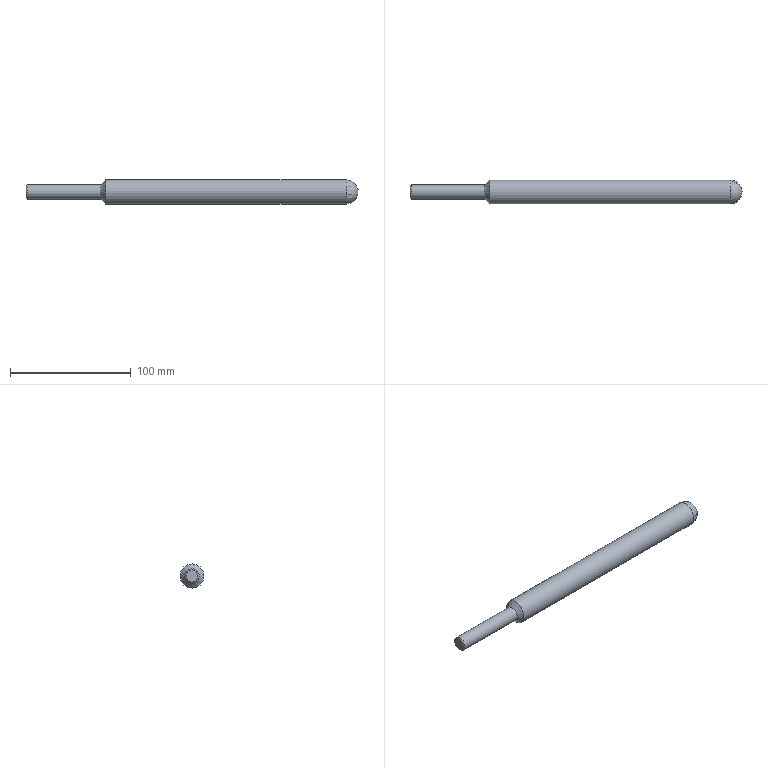Component | NX | TOMMY_BAR | 1 solid | 6 faces | box 275 x 20 x 20 mm | volume 72427 mm3 | cylinder 2 | cone 2 | plane 1 | sphere 1 | commonest cylinder face diameters 12 x1 20 x1
STEP:
#1=CARTESIAN_POINT('',(0.,0.,0.));
#2=DIRECTION('',(0.,0.,1.));
#3=DIRECTION('',(1.,0.,0.));
#4=AXIS2_PLACEMENT_3D('',#1,#2,#3);
#5=CARTESIAN_POINT('',(-19.,240.,259.5));
#6=VERTEX_POINT('',#5);
#7=CARTESIAN_POINT('',(-19.,246.,265.5));
#8=VERTEX_POINT('',#7);
#9=CARTESIAN_POINT('',(-19.,240.,265.5));
#10=DIRECTION('',(1.,0.,0.));
#11=DIRECTION('',(0.,0.,-1.));
#12=AXIS2_PLACEMENT_3D('',#9,#10,#11);
#13=CIRCLE('',#12,6.);
#14=CARTESIAN_POINT('',(42.,240.,265.5));
#15=DIRECTION('',(-1.,0.,0.));
#16=DIRECTION('',(0.,0.,1.));
#17=AXIS2_PLACEMENT_3D('',#14,#15,#16);
#18=CYLINDRICAL_SURFACE('',#17,6.);
#19=CARTESIAN_POINT('',(3.142,61.));
#20=DIRECTION('',(-1.,0.));
#21=VECTOR('',#20,1.);
#22=LINE('',#19,#21);
#23=(GEOMETRIC_REPRESENTATION_CONTEXT(2)PARAMETRIC_REPRESENTATION_CONTEXT()REPRESENTATION_CONTEXT('',''));
#24=DEFINITIONAL_REPRESENTATION('',(#22),#23);
#25=PCURVE('',#18,#24);
#26=CARTESIAN_POINT('',(-19.,240.,265.5));
#27=DIRECTION('',(1.,0.,0.));
#28=DIRECTION('',(0.,0.,-1.));
#29=AXIS2_PLACEMENT_3D('',#26,#27,#28);
#30=CONICAL_SURFACE('',#29,6.,0.7854);
#31=CARTESIAN_POINT('',(0.,0.));
#32=DIRECTION('',(1.,0.));
#33=VECTOR('',#32,1.);
#34=LINE('',#31,#33);
#35=(GEOMETRIC_REPRESENTATION_CONTEXT(2)PARAMETRIC_REPRESENTATION_CONTEXT()REPRESENTATION_CONTEXT('',''));
#36=DEFINITIONAL_REPRESENTATION('',(#34),#35);
#37=PCURVE('',#30,#36);
#38=SURFACE_CURVE('',#13,(#25,#37),.PCURVE_S1.);
#39=EDGE_CURVE('',#6,#8,#38,.T.);
#40=ORIENTED_EDGE('',*,*,#39,.T.);
#41=CARTESIAN_POINT('',(42.,246.,265.5));
#42=VERTEX_POINT('',#41);
#43=CARTESIAN_POINT('',(42.,246.,265.5));
#44=CARTESIAN_POINT('',(-19.,246.,265.5));
#45=B_SPLINE_CURVE_WITH_KNOTS('',1,(#43,#44),.UNSPECIFIED.,.F.,.F.,(2,2),(0.,61.),.PIECEWISE_BEZIER_KNOTS.);
#46=CARTESIAN_POINT('',(1.571,0.));
#47=DIRECTION('',(0.,1.));
#48=VECTOR('',#47,1.);
#49=LINE('',#46,#48);
#50=(GEOMETRIC_REPRESENTATION_CONTEXT(2)PARAMETRIC_REPRESENTATION_CONTEXT()REPRESENTATION_CONTEXT('',''));
#51=DEFINITIONAL_REPRESENTATION('',(#49),#50);
#52=PCURVE('',#18,#51);
#53=CARTESIAN_POINT('',(7.854,0.));
#54=DIRECTION('',(0.,1.));
#55=VECTOR('',#54,1.);
#56=LINE('',#53,#55);
#57=(GEOMETRIC_REPRESENTATION_CONTEXT(2)PARAMETRIC_REPRESENTATION_CONTEXT()REPRESENTATION_CONTEXT('',''));
#58=DEFINITIONAL_REPRESENTATION('',(#56),#57);
#59=PCURVE('',#18,#58);
#60=SEAM_CURVE('',#45,(#52,#59),.PCURVE_S1.);
#61=EDGE_CURVE('',#42,#8,#60,.T.);
#62=ORIENTED_EDGE('',*,*,#61,.F.);
#63=CARTESIAN_POINT('',(42.,240.,259.5));
#64=VERTEX_POINT('',#63);
#65=CARTESIAN_POINT('',(42.,240.,265.5));
#66=DIRECTION('',(1.,0.,0.));
#67=DIRECTION('',(0.,1.,0.));
#68=AXIS2_PLACEMENT_3D('',#65,#66,#67);
#69=CIRCLE('',#68,6.);
#70=CARTESIAN_POINT('',(7.854,0.));
#71=DIRECTION('',(-1.,0.));
#72=VECTOR('',#71,1.);
#73=LINE('',#70,#72);
#74=(GEOMETRIC_REPRESENTATION_CONTEXT(2)PARAMETRIC_REPRESENTATION_CONTEXT()REPRESENTATION_CONTEXT('',''));
#75=DEFINITIONAL_REPRESENTATION('',(#73),#74);
#76=PCURVE('',#18,#75);
#77=CARTESIAN_POINT('',(46.,240.,265.5));
#78=DIRECTION('',(1.,0.,0.));
#79=DIRECTION('',(0.,0.,-1.));
#80=AXIS2_PLACEMENT_3D('',#77,#78,#79);
#81=CONICAL_SURFACE('',#80,10.,0.7854);
#82=CARTESIAN_POINT('',(-4.712,-4.));
#83=DIRECTION('',(1.,0.));
#84=VECTOR('',#83,1.);
#85=LINE('',#82,#84);
#86=(GEOMETRIC_REPRESENTATION_CONTEXT(2)PARAMETRIC_REPRESENTATION_CONTEXT()REPRESENTATION_CONTEXT('',''));
#87=DEFINITIONAL_REPRESENTATION('',(#85),#86);
#88=PCURVE('',#81,#87);
#89=SURFACE_CURVE('',#69,(#76,#88),.PCURVE_S1.);
#90=EDGE_CURVE('',#64,#42,#89,.T.);
#91=ORIENTED_EDGE('',*,*,#90,.F.);
#92=CARTESIAN_POINT('',(42.,240.,265.5));
#93=DIRECTION('',(1.,0.,0.));
#94=DIRECTION('',(0.,1.,0.));
#95=AXIS2_PLACEMENT_3D('',#92,#93,#94);
#96=CIRCLE('',#95,6.);
#97=CARTESIAN_POINT('',(7.854,0.));
#98=DIRECTION('',(-1.,0.));
#99=VECTOR('',#98,1.);
#100=LINE('',#97,#99);
#101=(GEOMETRIC_REPRESENTATION_CONTEXT(2)PARAMETRIC_REPRESENTATION_CONTEXT()REPRESENTATION_CONTEXT('',''));
#102=DEFINITIONAL_REPRESENTATION('',(#100),#101);
#103=PCURVE('',#18,#102);
#104=CARTESIAN_POINT('',(1.571,-4.));
#105=DIRECTION('',(1.,0.));
#106=VECTOR('',#105,1.);
#107=LINE('',#104,#106);
#108=(GEOMETRIC_REPRESENTATION_CONTEXT(2)PARAMETRIC_REPRESENTATION_CONTEXT()REPRESENTATION_CONTEXT('',''));
#109=DEFINITIONAL_REPRESENTATION('',(#107),#108);
#110=PCURVE('',#81,#109);
#111=SURFACE_CURVE('',#96,(#103,#110),.PCURVE_S1.);
#112=EDGE_CURVE('',#42,#64,#111,.T.);
#113=ORIENTED_EDGE('',*,*,#112,.F.);
#114=ORIENTED_EDGE('',*,*,#61,.T.);
#115=CARTESIAN_POINT('',(-19.,240.,265.5));
#116=DIRECTION('',(1.,0.,0.));
#117=DIRECTION('',(0.,0.,-1.));
#118=AXIS2_PLACEMENT_3D('',#115,#116,#117);
#119=CIRCLE('',#118,6.);
#120=CARTESIAN_POINT('',(9.425,61.));
#121=DIRECTION('',(-1.,0.));
#122=VECTOR('',#121,1.);
#123=LINE('',#120,#122);
#124=(GEOMETRIC_REPRESENTATION_CONTEXT(2)PARAMETRIC_REPRESENTATION_CONTEXT()REPRESENTATION_CONTEXT('',''));
#125=DEFINITIONAL_REPRESENTATION('',(#123),#124);
#126=PCURVE('',#18,#125);
#127=CARTESIAN_POINT('',(0.,0.));
#128=DIRECTION('',(1.,0.));
#129=VECTOR('',#128,1.);
#130=LINE('',#127,#129);
#131=(GEOMETRIC_REPRESENTATION_CONTEXT(2)PARAMETRIC_REPRESENTATION_CONTEXT()REPRESENTATION_CONTEXT('',''));
#132=DEFINITIONAL_REPRESENTATION('',(#130),#131);
#133=PCURVE('',#30,#132);
#134=SURFACE_CURVE('',#119,(#126,#133),.PCURVE_S1.);
#135=EDGE_CURVE('',#8,#6,#134,.T.);
#136=ORIENTED_EDGE('',*,*,#135,.T.);
#137=EDGE_LOOP('',(#40,#62,#91,#113,#114,#136));
#138=FACE_BOUND('',#137,.T.);
#139=ADVANCED_FACE('',(#138),#18,.T.);
#140=CARTESIAN_POINT('',(-20.,240.,260.5));
#141=VERTEX_POINT('',#140);
#142=CARTESIAN_POINT('',(-20.,240.,265.5));
#143=DIRECTION('',(-1.,0.,0.));
#144=DIRECTION('',(0.,0.,-1.));
#145=AXIS2_PLACEMENT_3D('',#142,#143,#144);
#146=CIRCLE('',#145,5.);
#147=CARTESIAN_POINT('',(-20.,240.,265.5));
#148=DIRECTION('',(1.,0.,0.));
#149=DIRECTION('',(0.,0.,-1.));
#150=AXIS2_PLACEMENT_3D('',#147,#148,#149);
#151=PLANE('',#150);
#152=CARTESIAN_POINT('',(5.,0.));
#153=CARTESIAN_POINT('',(5.,-8.66));
#154=CARTESIAN_POINT('',(-2.5,-4.33));
#155=CARTESIAN_POINT('',(-10.,-0.));
#156=CARTESIAN_POINT('',(-2.5,4.33));
#157=CARTESIAN_POINT('',(5.,8.66));
#158=CARTESIAN_POINT('',(5.,0.));
#159=(BOUNDED_CURVE()B_SPLINE_CURVE(2,(#152,#153,#154,#155,#156,#157,#158),.UNSPECIFIED.,.T.,.F.)B_SPLINE_CURVE_WITH_KNOTS((1,2,2,2,2,1),(-2.094,0.,2.094,4.189,6.283,8.378),.UNSPECIFIED.)CURVE()GEOMETRIC_REPRESENTATION_ITEM()RATIONAL_B_SPLINE_CURVE((1.,0.5,1.,0.5,1.,0.5,1.))REPRESENTATION_ITEM(''));
#160=(GEOMETRIC_REPRESENTATION_CONTEXT(2)PARAMETRIC_REPRESENTATION_CONTEXT()REPRESENTATION_CONTEXT('',''));
#161=DEFINITIONAL_REPRESENTATION('',(#159),#160);
#162=PCURVE('',#151,#161);
#163=CARTESIAN_POINT('',(6.283,-1.));
#164=DIRECTION('',(-1.,0.));
#165=VECTOR('',#164,1.);
#166=LINE('',#163,#165);
#167=(GEOMETRIC_REPRESENTATION_CONTEXT(2)PARAMETRIC_REPRESENTATION_CONTEXT()REPRESENTATION_CONTEXT('',''));
#168=DEFINITIONAL_REPRESENTATION('',(#166),#167);
#169=PCURVE('',#30,#168);
#170=SURFACE_CURVE('',#146,(#162,#169),.PCURVE_S1.);
#171=EDGE_CURVE('',#141,#141,#170,.T.);
#172=ORIENTED_EDGE('',*,*,#171,.T.);
#173=EDGE_LOOP('',(#172));
#174=FACE_BOUND('',#173,.T.);
#175=ADVANCED_FACE('',(#174),#151,.F.);
#176=CARTESIAN_POINT('',(245.,240.,255.5));
#177=VERTEX_POINT('',#176);
#178=CARTESIAN_POINT('',(245.,240.,275.5));
#179=VERTEX_POINT('',#178);
#180=CARTESIAN_POINT('',(245.,240.,265.5));
#181=DIRECTION('',(-1.,0.,0.));
#182=DIRECTION('',(0.,0.,1.));
#183=AXIS2_PLACEMENT_3D('',#180,#181,#182);
#184=CIRCLE('',#183,10.);
#185=CARTESIAN_POINT('',(255.,240.,265.5));
#186=DIRECTION('',(-1.,0.,0.));
#187=DIRECTION('',(0.,0.,1.));
#188=AXIS2_PLACEMENT_3D('',#185,#186,#187);
#189=CYLINDRICAL_SURFACE('',#188,10.);
#190=CARTESIAN_POINT('',(0.,10.));
#191=DIRECTION('',(1.,0.));
#192=VECTOR('',#191,1.);
#193=LINE('',#190,#192);
#194=(GEOMETRIC_REPRESENTATION_CONTEXT(2)PARAMETRIC_REPRESENTATION_CONTEXT()REPRESENTATION_CONTEXT('',''));
#195=DEFINITIONAL_REPRESENTATION('',(#193),#194);
#196=PCURVE('',#189,#195);
#197=CARTESIAN_POINT('',(245.,240.,265.5));
#198=DIRECTION('',(0.,0.,1.));
#199=DIRECTION('',(1.,0.,0.));
#200=AXIS2_PLACEMENT_3D('',#197,#198,#199);
#201=SPHERICAL_SURFACE('',#200,10.);
#202=CARTESIAN_POINT('',(4.712,-1.571));
#203=CARTESIAN_POINT('',(4.712,-1.523));
#204=CARTESIAN_POINT('',(4.712,-1.428));
#205=CARTESIAN_POINT('',(4.712,-1.285));
#206=CARTESIAN_POINT('',(4.712,-1.142));
#207=CARTESIAN_POINT('',(4.712,-0.9996));
#208=CARTESIAN_POINT('',(4.712,-0.8568));
#209=CARTESIAN_POINT('',(4.712,-0.714));
#210=CARTESIAN_POINT('',(4.712,-0.5712));
#211=CARTESIAN_POINT('',(4.712,-0.4284));
#212=CARTESIAN_POINT('',(4.712,-0.2856));
#213=CARTESIAN_POINT('',(4.712,-0.1428));
#214=CARTESIAN_POINT('',(4.712,0.));
#215=CARTESIAN_POINT('',(4.712,0.1428));
#216=CARTESIAN_POINT('',(4.712,0.2856));
#217=CARTESIAN_POINT('',(4.712,0.4284));
#218=CARTESIAN_POINT('',(4.712,0.5712));
#219=CARTESIAN_POINT('',(4.712,0.714));
#220=CARTESIAN_POINT('',(4.712,0.8568));
#221=CARTESIAN_POINT('',(4.712,0.9996));
#222=CARTESIAN_POINT('',(4.712,1.142));
#223=CARTESIAN_POINT('',(4.712,1.285));
#224=CARTESIAN_POINT('',(4.712,1.428));
#225=CARTESIAN_POINT('',(4.712,1.523));
#226=CARTESIAN_POINT('',(4.712,1.571));
#227=B_SPLINE_CURVE_WITH_KNOTS('',3,(#202,#203,#204,#205,#206,#207,#208,#209,#210,#211,#212,#213,#214,#215,#216,#217,#218,#219,#220,#221,#222,#223,#224,#225,#226),.UNSPECIFIED.,.F.,.F.,(4,1,1,1,1,1,1,1,1,1,1,1,1,1,1,1,1,1,1,1,1,1,4),(3.142,3.284,3.427,3.57,3.713,3.856,3.998,4.141,4.284,4.427,4.57,4.712,4.855,4.998,5.141,5.284,5.426,5.569,5.712,5.855,5.998,6.14,6.283),.QUASI_UNIFORM_KNOTS.);
#228=(GEOMETRIC_REPRESENTATION_CONTEXT(2)PARAMETRIC_REPRESENTATION_CONTEXT()REPRESENTATION_CONTEXT('',''));
#229=DEFINITIONAL_REPRESENTATION('',(#227),#228);
#230=PCURVE('',#201,#229);
#231=SURFACE_CURVE('',#184,(#196,#230),.PCURVE_S1.);
#232=EDGE_CURVE('',#177,#179,#231,.T.);
#233=ORIENTED_EDGE('',*,*,#232,.T.);
#234=CARTESIAN_POINT('',(46.,240.,275.5));
#235=VERTEX_POINT('',#234);
#236=CARTESIAN_POINT('',(245.,240.,275.5));
#237=CARTESIAN_POINT('',(46.,240.,275.5));
#238=B_SPLINE_CURVE_WITH_KNOTS('',1,(#236,#237),.UNSPECIFIED.,.F.,.F.,(2,2),(10.,209.),.PIECEWISE_BEZIER_KNOTS.);
#239=CARTESIAN_POINT('',(6.283,0.));
#240=DIRECTION('',(0.,1.));
#241=VECTOR('',#240,1.);
#242=LINE('',#239,#241);
#243=(GEOMETRIC_REPRESENTATION_CONTEXT(2)PARAMETRIC_REPRESENTATION_CONTEXT()REPRESENTATION_CONTEXT('',''));
#244=DEFINITIONAL_REPRESENTATION('',(#242),#243);
#245=PCURVE('',#189,#244);
#246=CARTESIAN_POINT('',(0.,0.));
#247=DIRECTION('',(0.,1.));
#248=VECTOR('',#247,1.);
#249=LINE('',#246,#248);
#250=(GEOMETRIC_REPRESENTATION_CONTEXT(2)PARAMETRIC_REPRESENTATION_CONTEXT()REPRESENTATION_CONTEXT('',''));
#251=DEFINITIONAL_REPRESENTATION('',(#249),#250);
#252=PCURVE('',#189,#251);
#253=SEAM_CURVE('',#238,(#245,#252),.PCURVE_S1.);
#254=EDGE_CURVE('',#179,#235,#253,.T.);
#255=ORIENTED_EDGE('',*,*,#254,.T.);
#256=CARTESIAN_POINT('',(46.,240.,255.5));
#257=VERTEX_POINT('',#256);
#258=CARTESIAN_POINT('',(46.,240.,265.5));
#259=DIRECTION('',(1.,0.,0.));
#260=DIRECTION('',(0.,0.,-1.));
#261=AXIS2_PLACEMENT_3D('',#258,#259,#260);
#262=CIRCLE('',#261,10.);
#263=CARTESIAN_POINT('',(9.425,209.));
#264=DIRECTION('',(-1.,0.));
#265=VECTOR('',#264,1.);
#266=LINE('',#263,#265);
#267=(GEOMETRIC_REPRESENTATION_CONTEXT(2)PARAMETRIC_REPRESENTATION_CONTEXT()REPRESENTATION_CONTEXT('',''));
#268=DEFINITIONAL_REPRESENTATION('',(#266),#267);
#269=PCURVE('',#189,#268);
#270=CARTESIAN_POINT('',(0.,0.));
#271=DIRECTION('',(1.,0.));
#272=VECTOR('',#271,1.);
#273=LINE('',#270,#272);
#274=(GEOMETRIC_REPRESENTATION_CONTEXT(2)PARAMETRIC_REPRESENTATION_CONTEXT()REPRESENTATION_CONTEXT('',''));
#275=DEFINITIONAL_REPRESENTATION('',(#273),#274);
#276=PCURVE('',#81,#275);
#277=SURFACE_CURVE('',#262,(#269,#276),.PCURVE_S1.);
#278=EDGE_CURVE('',#235,#257,#277,.T.);
#279=ORIENTED_EDGE('',*,*,#278,.T.);
#280=CARTESIAN_POINT('',(46.,240.,265.5));
#281=DIRECTION('',(1.,0.,0.));
#282=DIRECTION('',(0.,0.,-1.));
#283=AXIS2_PLACEMENT_3D('',#280,#281,#282);
#284=CIRCLE('',#283,10.);
#285=CARTESIAN_POINT('',(3.142,209.));
#286=DIRECTION('',(-1.,0.));
#287=VECTOR('',#286,1.);
#288=LINE('',#285,#287);
#289=(GEOMETRIC_REPRESENTATION_CONTEXT(2)PARAMETRIC_REPRESENTATION_CONTEXT()REPRESENTATION_CONTEXT('',''));
#290=DEFINITIONAL_REPRESENTATION('',(#288),#289);
#291=PCURVE('',#189,#290);
#292=CARTESIAN_POINT('',(0.,0.));
#293=DIRECTION('',(1.,0.));
#294=VECTOR('',#293,1.);
#295=LINE('',#292,#294);
#296=(GEOMETRIC_REPRESENTATION_CONTEXT(2)PARAMETRIC_REPRESENTATION_CONTEXT()REPRESENTATION_CONTEXT('',''));
#297=DEFINITIONAL_REPRESENTATION('',(#295),#296);
#298=PCURVE('',#81,#297);
#299=SURFACE_CURVE('',#284,(#291,#298),.PCURVE_S1.);
#300=EDGE_CURVE('',#257,#235,#299,.T.);
#301=ORIENTED_EDGE('',*,*,#300,.T.);
#302=ORIENTED_EDGE('',*,*,#254,.F.);
#303=CARTESIAN_POINT('',(245.,240.,265.5));
#304=DIRECTION('',(-1.,0.,0.));
#305=DIRECTION('',(0.,0.,1.));
#306=AXIS2_PLACEMENT_3D('',#303,#304,#305);
#307=CIRCLE('',#306,10.);
#308=CARTESIAN_POINT('',(0.,10.));
#309=DIRECTION('',(1.,0.));
#310=VECTOR('',#309,1.);
#311=LINE('',#308,#310);
#312=(GEOMETRIC_REPRESENTATION_CONTEXT(2)PARAMETRIC_REPRESENTATION_CONTEXT()REPRESENTATION_CONTEXT('',''));
#313=DEFINITIONAL_REPRESENTATION('',(#311),#312);
#314=PCURVE('',#189,#313);
#315=CARTESIAN_POINT('',(7.854,1.571));
#316=CARTESIAN_POINT('',(7.854,1.523));
#317=CARTESIAN_POINT('',(7.854,1.428));
#318=CARTESIAN_POINT('',(7.854,1.285));
#319=CARTESIAN_POINT('',(7.854,1.142));
#320=CARTESIAN_POINT('',(7.854,0.9996));
#321=CARTESIAN_POINT('',(7.854,0.8568));
#322=CARTESIAN_POINT('',(7.854,0.714));
#323=CARTESIAN_POINT('',(7.854,0.5712));
#324=CARTESIAN_POINT('',(7.854,0.4284));
#325=CARTESIAN_POINT('',(7.854,0.2856));
#326=CARTESIAN_POINT('',(7.854,0.1428));
#327=CARTESIAN_POINT('',(7.854,0.));
#328=CARTESIAN_POINT('',(7.854,-0.1428));
#329=CARTESIAN_POINT('',(7.854,-0.2856));
#330=CARTESIAN_POINT('',(7.854,-0.4284));
#331=CARTESIAN_POINT('',(7.854,-0.5712));
#332=CARTESIAN_POINT('',(7.854,-0.714));
#333=CARTESIAN_POINT('',(7.854,-0.8568));
#334=CARTESIAN_POINT('',(7.854,-0.9996));
#335=CARTESIAN_POINT('',(7.854,-1.142));
#336=CARTESIAN_POINT('',(7.854,-1.285));
#337=CARTESIAN_POINT('',(7.854,-1.428));
#338=CARTESIAN_POINT('',(7.854,-1.523));
#339=CARTESIAN_POINT('',(7.854,-1.571));
#340=B_SPLINE_CURVE_WITH_KNOTS('',3,(#315,#316,#317,#318,#319,#320,#321,#322,#323,#324,#325,#326,#327,#328,#329,#330,#331,#332,#333,#334,#335,#336,#337,#338,#339),.UNSPECIFIED.,.F.,.F.,(4,1,1,1,1,1,1,1,1,1,1,1,1,1,1,1,1,1,1,1,1,1,4),(0.,0.1428,0.2856,0.4284,0.5712,0.714,0.8568,0.9996,1.142,1.285,1.428,1.571,1.714,1.856,1.999,2.142,2.285,2.428,2.57,2.713,2.856,2.999,3.142),.QUASI_UNIFORM_KNOTS.);
#341=(GEOMETRIC_REPRESENTATION_CONTEXT(2)PARAMETRIC_REPRESENTATION_CONTEXT()REPRESENTATION_CONTEXT('',''));
#342=DEFINITIONAL_REPRESENTATION('',(#340),#341);
#343=PCURVE('',#201,#342);
#344=SURFACE_CURVE('',#307,(#314,#343),.PCURVE_S1.);
#345=EDGE_CURVE('',#179,#177,#344,.T.);
#346=ORIENTED_EDGE('',*,*,#345,.T.);
#347=EDGE_LOOP('',(#233,#255,#279,#301,#302,#346));
#348=FACE_BOUND('',#347,.T.);
#349=ADVANCED_FACE('',(#348),#189,.T.);
#350=ORIENTED_EDGE('',*,*,#112,.T.);
#351=CARTESIAN_POINT('',(42.,240.,259.5));
#352=CARTESIAN_POINT('',(46.,240.,255.5));
#353=B_SPLINE_CURVE_WITH_KNOTS('',1,(#351,#352),.UNSPECIFIED.,.F.,.F.,(2,2),(-5.657,0.),.PIECEWISE_BEZIER_KNOTS.);
#354=CARTESIAN_POINT('',(6.283,0.));
#355=DIRECTION('',(0.,1.));
#356=VECTOR('',#355,1.);
#357=LINE('',#354,#356);
#358=(GEOMETRIC_REPRESENTATION_CONTEXT(2)PARAMETRIC_REPRESENTATION_CONTEXT()REPRESENTATION_CONTEXT('',''));
#359=DEFINITIONAL_REPRESENTATION('',(#357),#358);
#360=PCURVE('',#81,#359);
#361=CARTESIAN_POINT('',(0.,0.));
#362=DIRECTION('',(0.,1.));
#363=VECTOR('',#362,1.);
#364=LINE('',#361,#363);
#365=(GEOMETRIC_REPRESENTATION_CONTEXT(2)PARAMETRIC_REPRESENTATION_CONTEXT()REPRESENTATION_CONTEXT('',''));
#366=DEFINITIONAL_REPRESENTATION('',(#364),#365);
#367=PCURVE('',#81,#366);
#368=SEAM_CURVE('',#353,(#360,#367),.PCURVE_S1.);
#369=EDGE_CURVE('',#64,#257,#368,.T.);
#370=ORIENTED_EDGE('',*,*,#369,.T.);
#371=ORIENTED_EDGE('',*,*,#278,.F.);
#372=ORIENTED_EDGE('',*,*,#300,.F.);
#373=ORIENTED_EDGE('',*,*,#369,.F.);
#374=ORIENTED_EDGE('',*,*,#90,.T.);
#375=EDGE_LOOP('',(#350,#370,#371,#372,#373,#374));
#376=FACE_BOUND('',#375,.T.);
#377=ADVANCED_FACE('',(#376),#81,.T.);
#378=ORIENTED_EDGE('',*,*,#171,.F.);
#379=CARTESIAN_POINT('',(-20.,240.,260.5));
#380=CARTESIAN_POINT('',(-19.,240.,259.5));
#381=B_SPLINE_CURVE_WITH_KNOTS('',1,(#379,#380),.UNSPECIFIED.,.F.,.F.,(2,2),(-1.414,0.),.PIECEWISE_BEZIER_KNOTS.);
#382=CARTESIAN_POINT('',(6.283,0.));
#383=DIRECTION('',(0.,1.));
#384=VECTOR('',#383,1.);
#385=LINE('',#382,#384);
#386=(GEOMETRIC_REPRESENTATION_CONTEXT(2)PARAMETRIC_REPRESENTATION_CONTEXT()REPRESENTATION_CONTEXT('',''));
#387=DEFINITIONAL_REPRESENTATION('',(#385),#386);
#388=PCURVE('',#30,#387);
#389=CARTESIAN_POINT('',(0.,0.));
#390=DIRECTION('',(0.,1.));
#391=VECTOR('',#390,1.);
#392=LINE('',#389,#391);
#393=(GEOMETRIC_REPRESENTATION_CONTEXT(2)PARAMETRIC_REPRESENTATION_CONTEXT()REPRESENTATION_CONTEXT('',''));
#394=DEFINITIONAL_REPRESENTATION('',(#392),#393);
#395=PCURVE('',#30,#394);
#396=SEAM_CURVE('',#381,(#388,#395),.PCURVE_S1.);
#397=EDGE_CURVE('',#141,#6,#396,.T.);
#398=ORIENTED_EDGE('',*,*,#397,.T.);
#399=ORIENTED_EDGE('',*,*,#135,.F.);
#400=ORIENTED_EDGE('',*,*,#39,.F.);
#401=ORIENTED_EDGE('',*,*,#397,.F.);
#402=EDGE_LOOP('',(#378,#398,#399,#400,#401));
#403=FACE_BOUND('',#402,.T.);
#404=ADVANCED_FACE('',(#403),#30,.T.);
#405=ORIENTED_EDGE('',*,*,#232,.F.);
#406=ORIENTED_EDGE('',*,*,#345,.F.);
#407=EDGE_LOOP('',(#405,#406));
#408=FACE_BOUND('',#407,.T.);
#409=ADVANCED_FACE('',(#408),#201,.T.);
#410=CLOSED_SHELL('',(#139,#175,#349,#377,#404,#409));
#411=MANIFOLD_SOLID_BREP('',#410);
#412=(LENGTH_UNIT()NAMED_UNIT(*)SI_UNIT(.MILLI.,.METRE.));
#413=UNCERTAINTY_MEASURE_WITH_UNIT(LENGTH_MEASURE(0.000005),#412,'','');
#414=(NAMED_UNIT(*)PLANE_ANGLE_UNIT()SI_UNIT($,.RADIAN.));
#415=(NAMED_UNIT(*)SI_UNIT($,.STERADIAN.)SOLID_ANGLE_UNIT());
#416=(GEOMETRIC_REPRESENTATION_CONTEXT(3)GLOBAL_UNCERTAINTY_ASSIGNED_CONTEXT((#413))GLOBAL_UNIT_ASSIGNED_CONTEXT((#412,#414,#415))REPRESENTATION_CONTEXT('',''));
#417=ADVANCED_BREP_SHAPE_REPRESENTATION('',(#4,#411),#416);